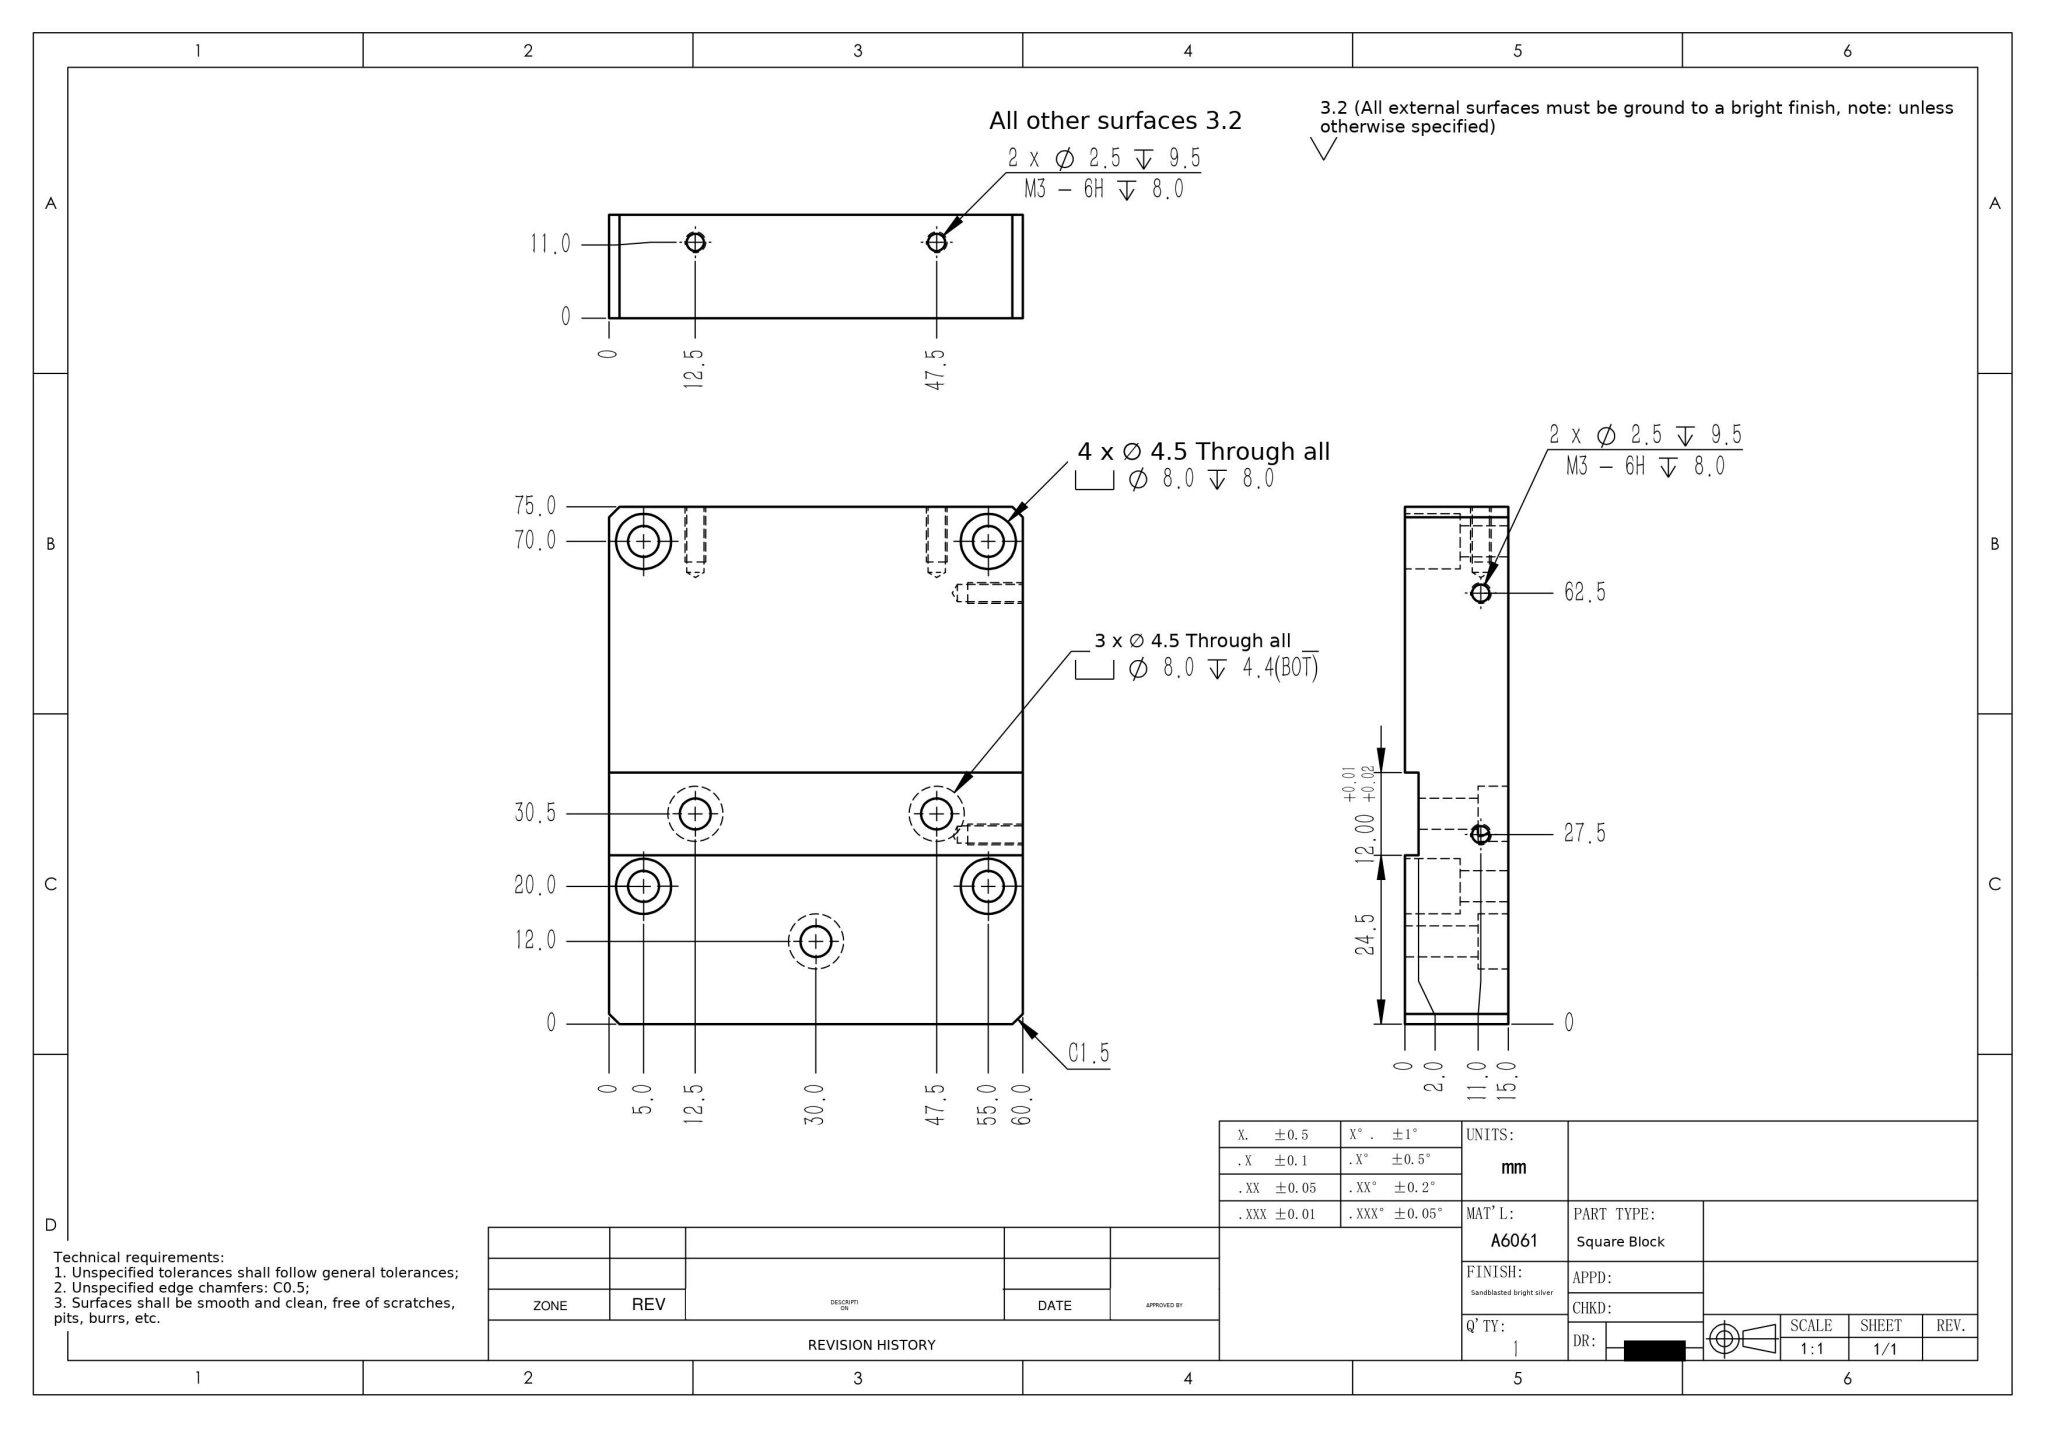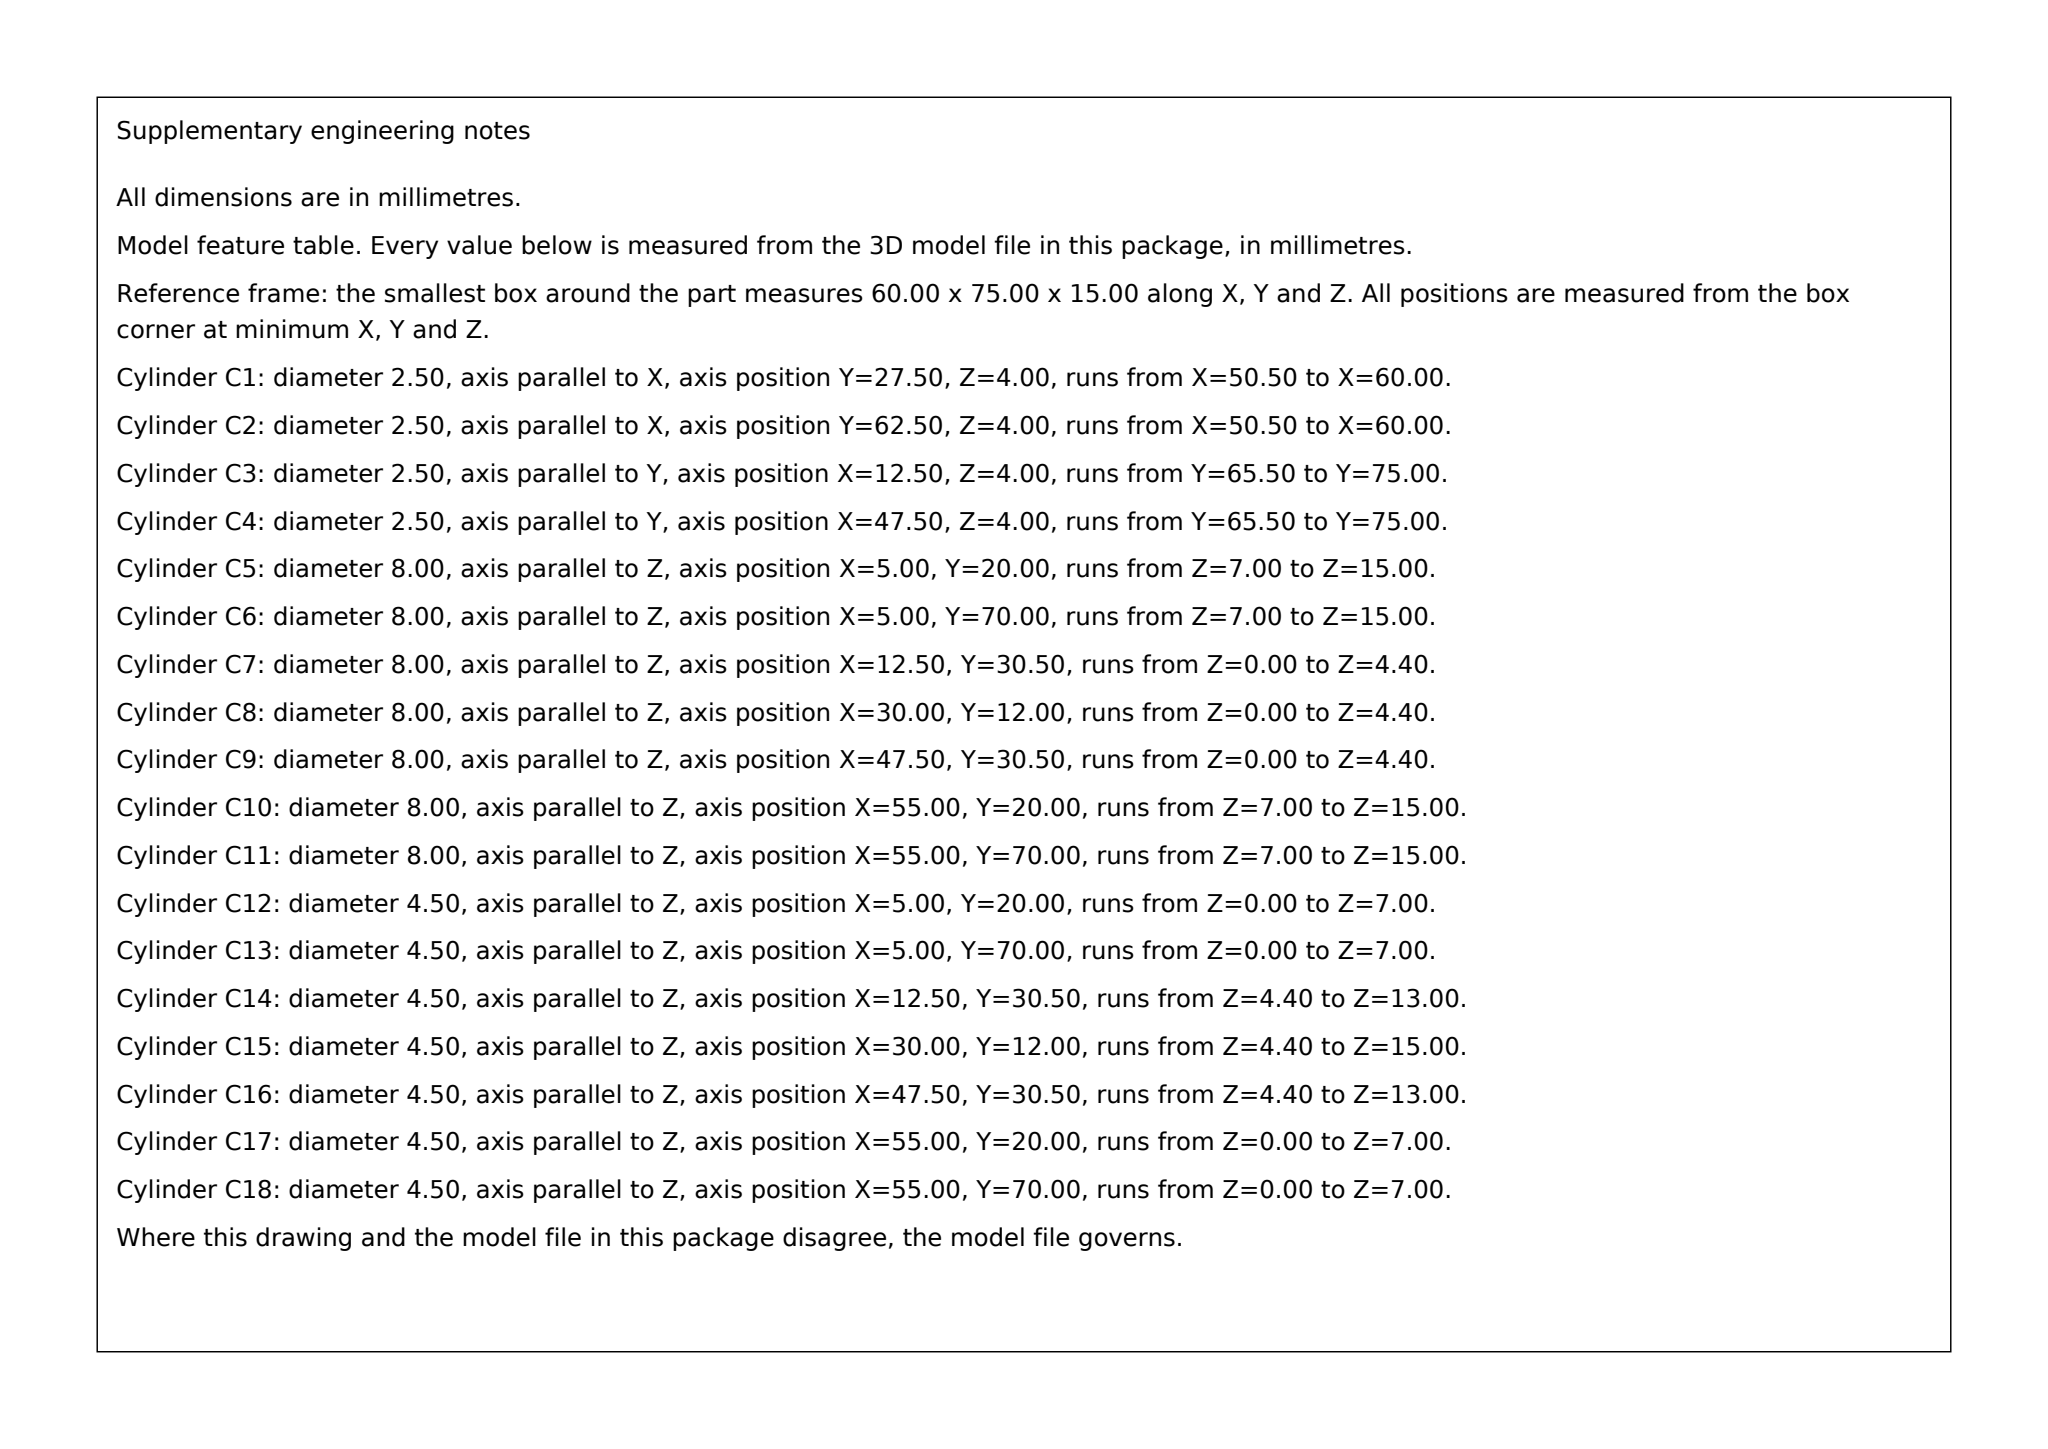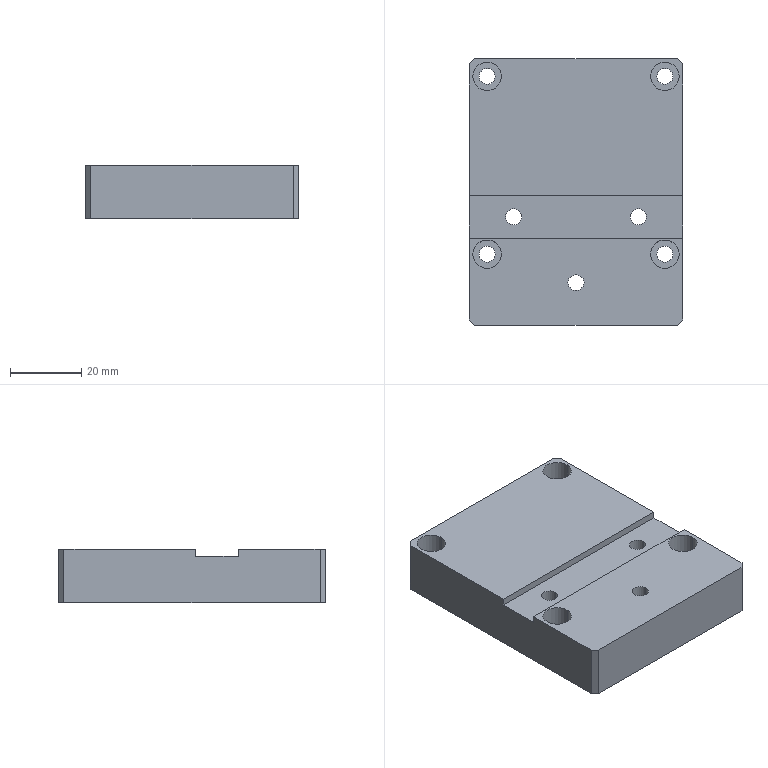Part | SolidWorks | mm | 1 solid | 66 faces | box 60 x 75 x 15 mm | volume 62642 mm3 | cylinder 36 | plane 21 | cone 9 | commonest cylinder face diameters 8 x14 4.5 x14 2.5 x8
build123d program:
from build123d import *

# Parameters (mm, degrees)
SKETCH1_W                                       = 60
SKETCH1_H                                       = 75
BOSS_EXTRUDE1_DEPTH                             = 15
SKETCH2_W                                       = 60
SKETCH2_H                                       = 12
CUT_EXTRUDE1_DEPTH                              = 2
M4_HEX_SOCKET_HEAD_CAP_SCREW_CBORE1_D           = 4.5
M4_HEX_SOCKET_HEAD_CAP_SCREW_CBORE1_CBORE_D     = 8
M4_HEX_SOCKET_HEAD_CAP_SCREW_CBORE1_CBORE_DEPTH = 8
M4_HEX_SOCKET_HEAD_CAP_SCREW_CBORE4_D           = 4.5
M4_HEX_SOCKET_HEAD_CAP_SCREW_CBORE4_CBORE_D     = 8
M4_HEX_SOCKET_HEAD_CAP_SCREW_CBORE4_CBORE_DEPTH = 4.4
M3_TAPPED_HOLE1_D                               = 2.5
M3_TAPPED_HOLE1_DEPTH                           = 9.5
M3_TAPPED_HOLE1_TIP                             = 0.7511
M3_TAPPED_HOLE2_D                               = 2.5
M3_TAPPED_HOLE2_DEPTH                           = 9.5
M3_TAPPED_HOLE2_TIP                             = 0.7511
CHAMFER1_SIZE                                   = 1.5


with BuildPart() as part:
    # Sketch1 → Boss-Extrude1 (new body)
    with BuildSketch(Plane.XY):
        with Locations((0, -37.5)):
            Rectangle(SKETCH1_W, SKETCH1_H)
    extrude(amount=BOSS_EXTRUDE1_DEPTH)

    # Sketch2 → Cut-Extrude1 (cut)
    with BuildSketch(Plane.XY.offset(15)):
        with Locations((0, -44.5)):
            Rectangle(SKETCH2_W, SKETCH2_H)
    extrude(amount=-CUT_EXTRUDE1_DEPTH, mode=Mode.SUBTRACT)

    # M4 Hex Socket Head Cap Screw CBORE1 (through all)
    with Locations(Plane.XY.offset(15)):
        with Locations((-25, -5), (25, -5), (25, -55), (-25, -55)):
            CounterBoreHole(M4_HEX_SOCKET_HEAD_CAP_SCREW_CBORE1_D / 2, M4_HEX_SOCKET_HEAD_CAP_SCREW_CBORE1_CBORE_D / 2, M4_HEX_SOCKET_HEAD_CAP_SCREW_CBORE1_CBORE_DEPTH)

    # M4 Hex Socket Head Cap Screw CBORE4 (through all)
    with Locations(Plane(origin=(0, 0, 0), x_dir=(-1, 0, 0), z_dir=(0, 0, -1))):
        with Locations((-17.5, -44.5), (17.5, -44.5), (0, -63)):
            CounterBoreHole(M4_HEX_SOCKET_HEAD_CAP_SCREW_CBORE4_D / 2, M4_HEX_SOCKET_HEAD_CAP_SCREW_CBORE4_CBORE_D / 2, M4_HEX_SOCKET_HEAD_CAP_SCREW_CBORE4_CBORE_DEPTH)

    # M3 Tapped Hole1
    with Locations(Plane(origin=(30, 0, 0), x_dir=(0, 0, -1), z_dir=(1, 0, 0))):
        with Locations((-4, -47.5), (-4, -12.5)):
            Hole(M3_TAPPED_HOLE1_D / 2, depth=M3_TAPPED_HOLE1_DEPTH)
            with Locations((0, 0, -(M3_TAPPED_HOLE1_DEPTH + M3_TAPPED_HOLE1_TIP / 2))):  # 118° drill point
                Cone(0, M3_TAPPED_HOLE1_D / 2, M3_TAPPED_HOLE1_TIP, mode=Mode.SUBTRACT)

    # M3 Tapped Hole2
    with Locations(Plane(origin=(0, 0, 0), x_dir=(1, 0, 0), z_dir=(0, 1, 0))):
        with Locations((17.5, -4), (-17.5, -4)):
            Hole(M3_TAPPED_HOLE2_D / 2, depth=M3_TAPPED_HOLE2_DEPTH)
            with Locations((0, 0, -(M3_TAPPED_HOLE2_DEPTH + M3_TAPPED_HOLE2_TIP / 2))):  # 118° drill point
                Cone(0, M3_TAPPED_HOLE2_D / 2, M3_TAPPED_HOLE2_TIP, mode=Mode.SUBTRACT)

    # Chamfer1
    chamfer1_edges = [part.edges().sort_by_distance(p)[0] for p in [
        (-30, 0, 7.5),
        (30, 0, 7.5),
        (30, -75, 7.5),
        (-30, -75, 7.5),
    ]]
    chamfer(chamfer1_edges, length=CHAMFER1_SIZE)


solid = part.part